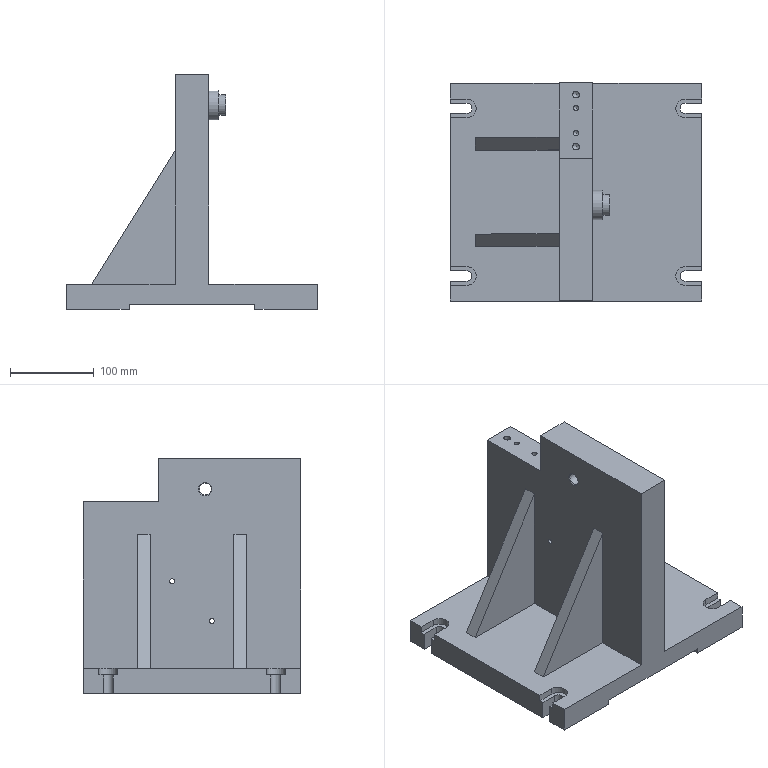Component | NX | FIXTURE_BODY | 1 solid | 83 faces | volume 4708238 mm3 | plane 49 | cylinder 22 | cone 12 | commonest cylinder face diameters 5.9 x4 6 x4 12 x4 22 x4 7.9 x2 35 x1 24.8 x1 20 x1